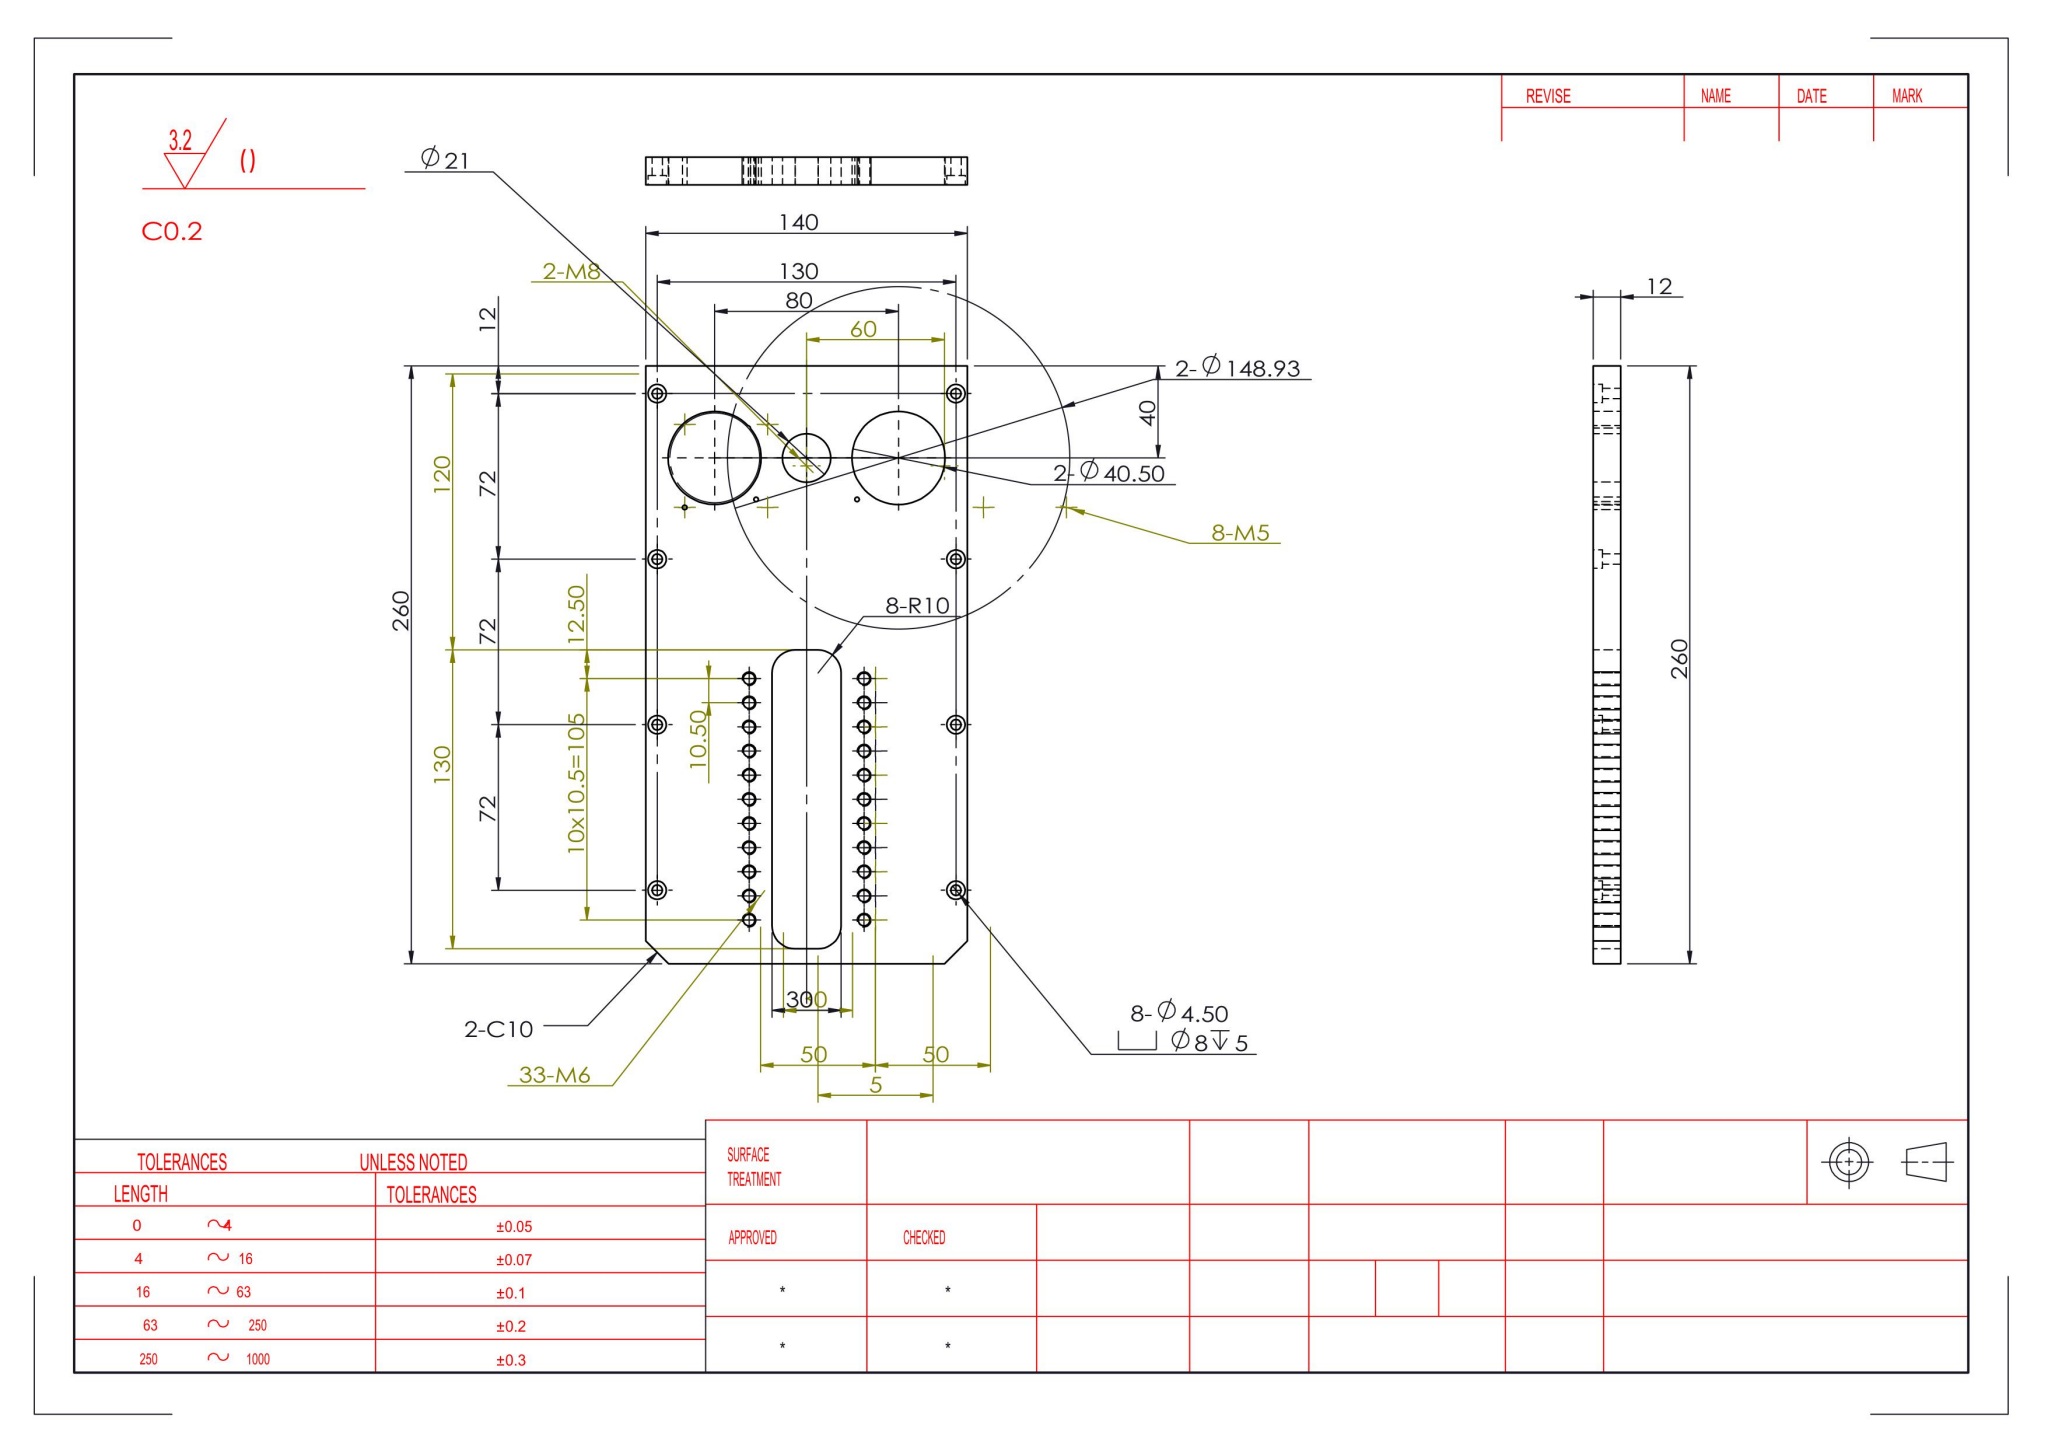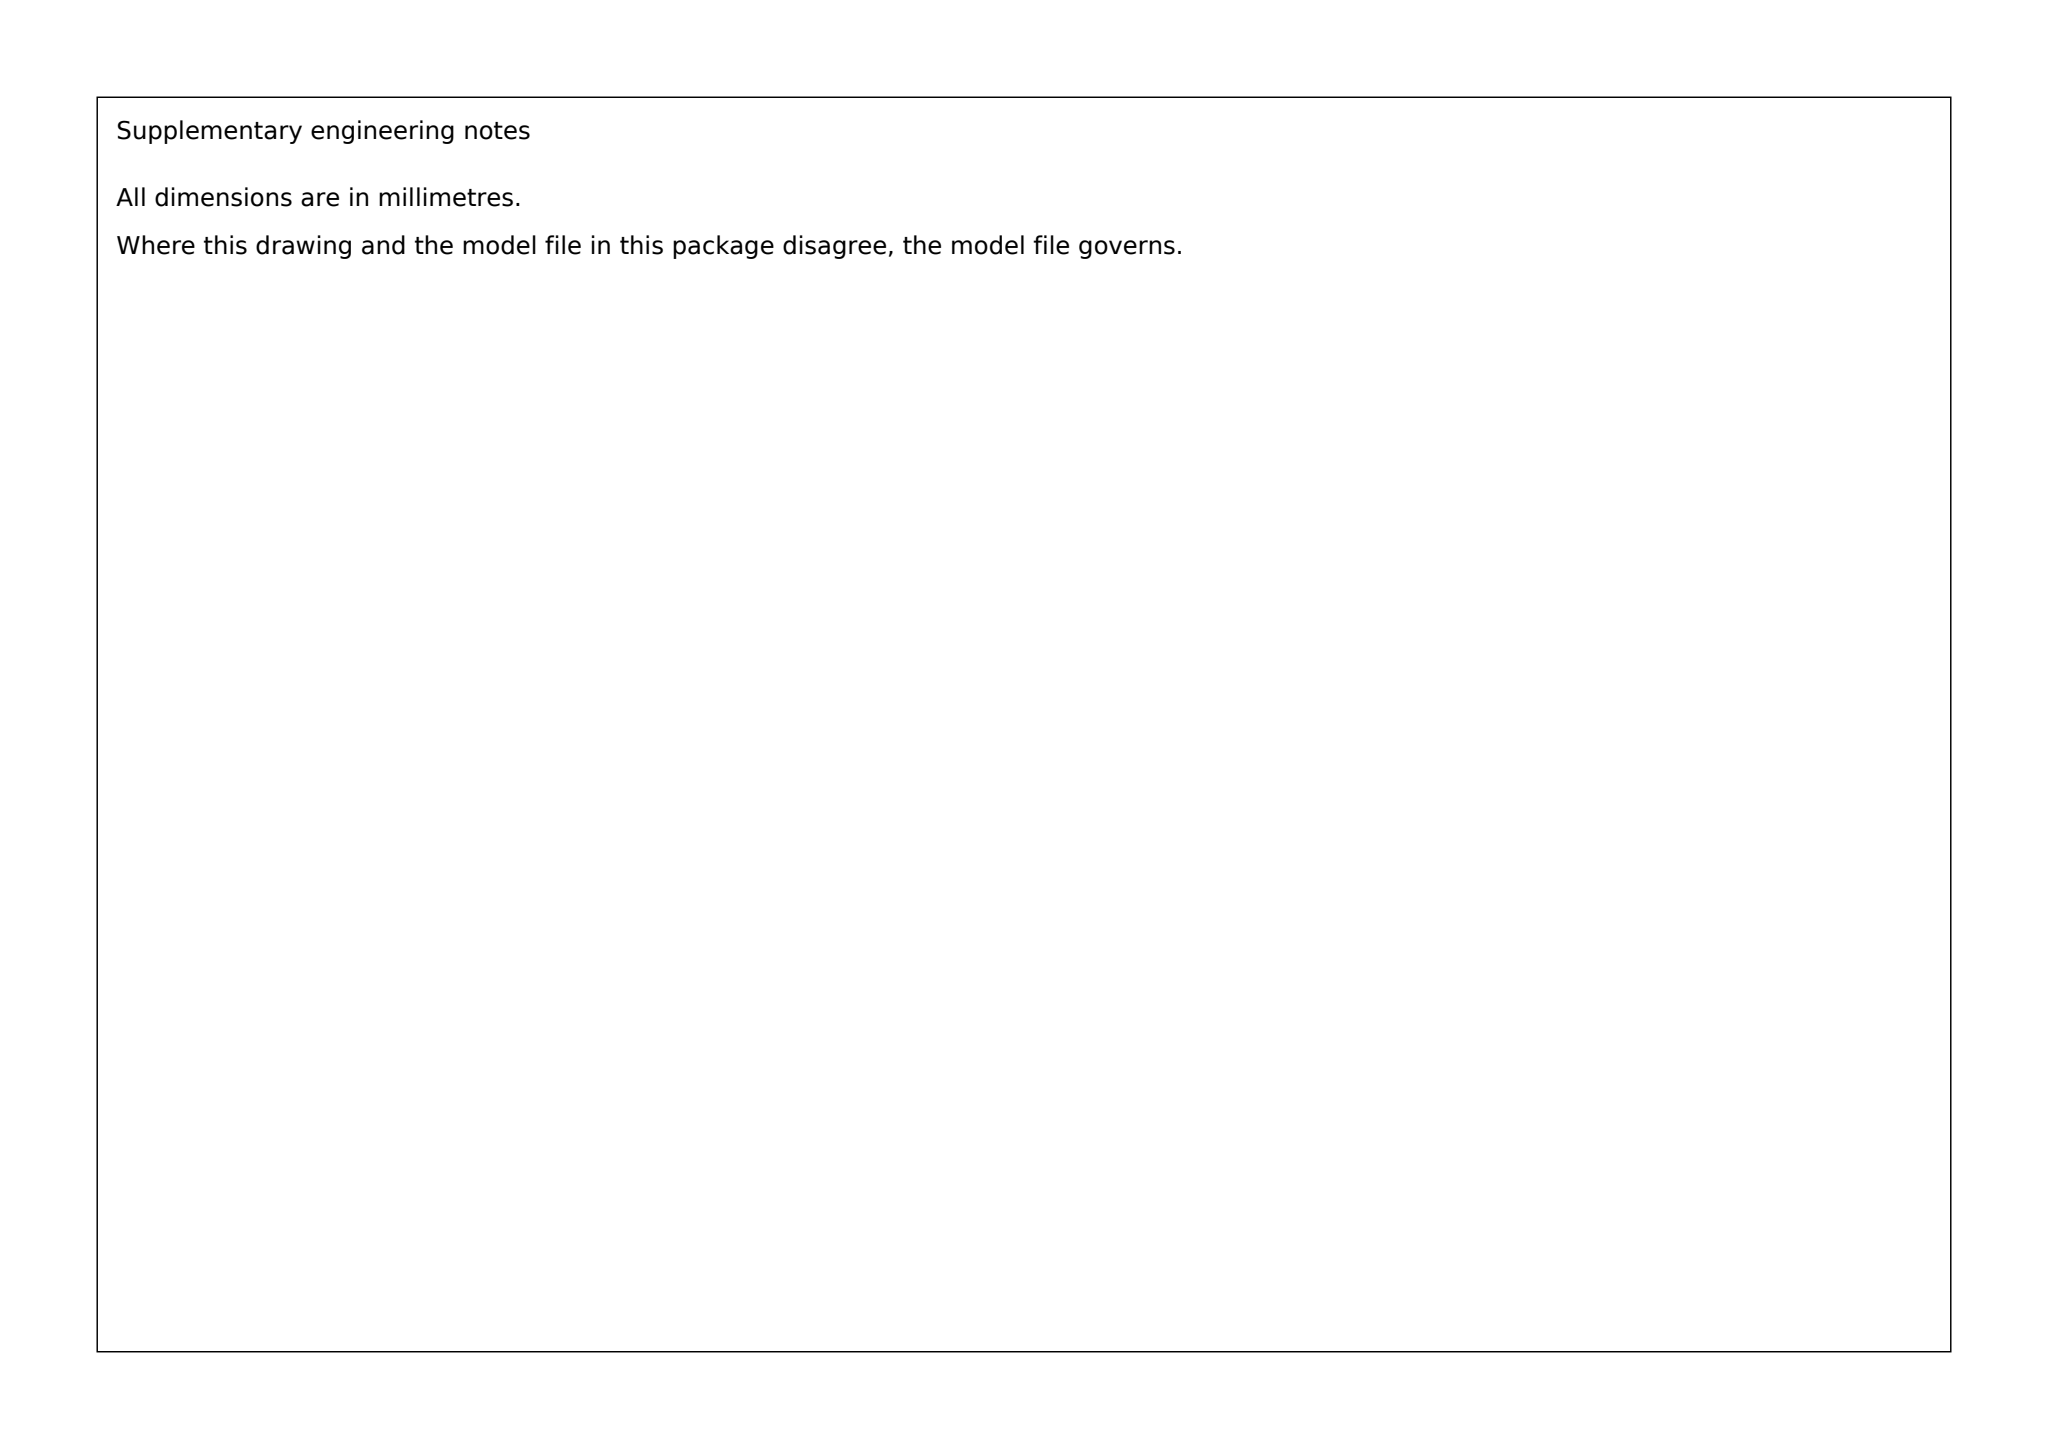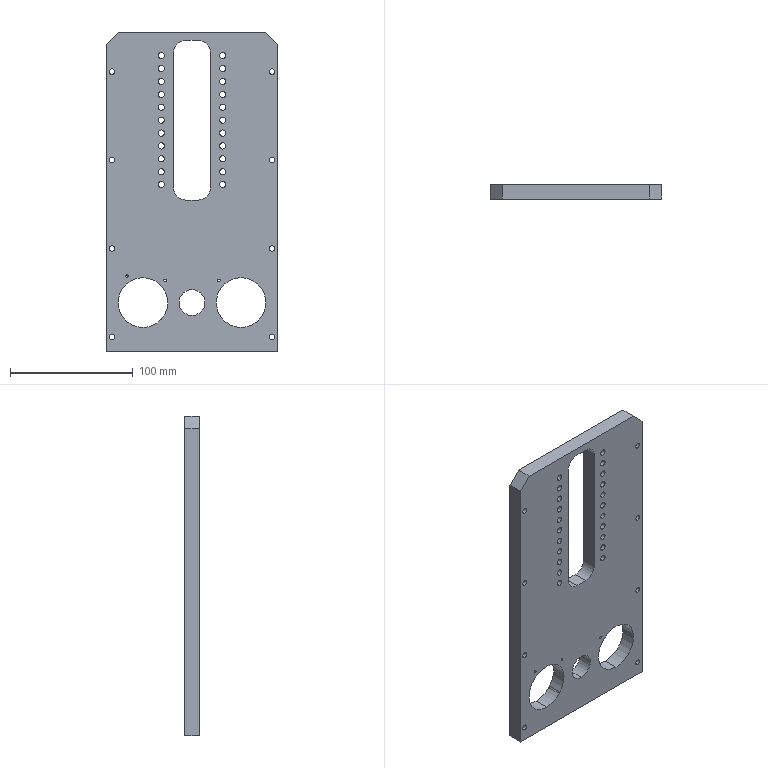Part | SolidWorks | mm | 1 solid | 114 faces | box 140 x 12 x 260 mm | volume 346829 mm3 | cylinder 94 | plane 20 | commonest cylinder face diameters 5 x44 8 x16 4.5 x16 2 x7 40.5 x5 20 x4 21 x2
build123d program:
from build123d import *

# Parameters (mm, degrees)
SKETCH1_W                                       = 140
SKETCH1_H                                       = 260
SKETCH1_R                                       = 20.25
SKETCH1_R_2                                     = 10.5
SKETCH1_W_2                                     = 30
SKETCH1_H_2                                     = 130
EXTRUDE1_DEPTH                                  = 12
CHAMFER1_SIZE                                   = 10
FILLET1_R                                       = 10
M6_TAPPED_HOLE1_D                               = 5
M4_HEX_SOCKET_HEAD_CAP_SCREW_CBORE1_D           = 4.5
M4_HEX_SOCKET_HEAD_CAP_SCREW_CBORE1_CBORE_D     = 8
M4_HEX_SOCKET_HEAD_CAP_SCREW_CBORE1_CBORE_DEPTH = 4
SKETCH5_R                                       = 1
EXTRUDE3_DEPTH                                  = 325.49


with BuildPart() as part:
    # Sketch1 → Extrude1 (new body)
    with BuildSketch(Plane(origin=(0, 0, 0), x_dir=(1, 0, 0), z_dir=(0, 1, 0))):
        with Locations((-19.315, 181.726)):
            Rectangle(SKETCH1_W, SKETCH1_H)
        with Locations(Location((-59.315, 271.726, 0), (0, 0, 270))):
            Circle(SKETCH1_R, mode=Mode.SUBTRACT)
        with Locations(Location((20.685, 271.726, 0), (0, 0, 270))):
            Circle(SKETCH1_R, mode=Mode.SUBTRACT)
        with Locations(Location((-19.315, 271.726, 0), (0, 0, 270))):
            Circle(SKETCH1_R_2, mode=Mode.SUBTRACT)
        with Locations((-19.315, 123.242)):
            Rectangle(SKETCH1_W_2, SKETCH1_H_2, mode=Mode.SUBTRACT)
    extrude(amount=EXTRUDE1_DEPTH)

    # Chamfer1
    chamfer1_edges = [part.edges().sort_by_distance(p)[0] for p in [
        (50.685, 6, -51.726),
        (-89.315, 6, -51.726),
    ]]
    chamfer(chamfer1_edges, length=CHAMFER1_SIZE)

    # Fillet1
    fillet1_edges = [part.edges().sort_by_distance(p)[0] for p in [
        (-34.315, 6, -58.242),
        (-4.315, 6, -58.242),
        (-4.315, 6, -188.242),
        (-34.315, 6, -188.242),
    ]]
    fillet(fillet1_edges, radius=FILLET1_R)

    # M6 Tapped Hole1 (through all)
    with Locations(Plane(origin=(5.685, 12, -70.742), x_dir=(0, 0, 1), z_dir=(0, 1, 0))):
        with Locations((0, 0), (-21, -50), (-42, 0), (-84, 0), (-105, -50), (-63, -50), (-84, -50), (-42, -50), (0, -50), (-21, 0), (-63, 0), (-105, 0), (-94.5, -50), (-73.5, -50), (-52.5, -50), (-31.5, -50), (-10.5, -50), (-94.5, 0), (-73.5, 0), (-52.5, 0), (-31.5, 0), (-10.5, 0)):
            Hole(M6_TAPPED_HOLE1_D / 2)

    # M4 Hex Socket Head Cap Screw CBORE1 (through all)
    with Locations(Plane(origin=(-84.315, 12, -299.726), x_dir=(0, 0, 1), z_dir=(0, 1, 0))):
        with Locations((0, 0), (72, 0), (144, 0), (216, 0), (0, 130), (72, 130), (144, 130), (216, 130)):
            CounterBoreHole(M4_HEX_SOCKET_HEAD_CAP_SCREW_CBORE1_D / 2, M4_HEX_SOCKET_HEAD_CAP_SCREW_CBORE1_CBORE_D / 2, M4_HEX_SOCKET_HEAD_CAP_SCREW_CBORE1_CBORE_DEPTH)

    # Sketch5 → Extrude3 (cut, through all)
    with BuildSketch(Plane(origin=(0, 12, 0), x_dir=(-1, 0, 0), z_dir=(0, 1, 0))):
        with Locations(Location((41.284, -253.694, 0), (0, 0, 90))):
            Circle(SKETCH5_R)
        with Locations(Location((-2.654, -253.694, 0), (0, 0, 90))):
            Circle(SKETCH5_R)
        with Locations(Location((72.346, -250.211, 0), (0, 0, 90))):
            Circle(SKETCH5_R)
        with Locations((75.83, -281.273)):
            Circle(SKETCH5_R)
        with Locations((44.767, -284.757)):
            Circle(SKETCH5_R)
    extrude(amount=-EXTRUDE3_DEPTH, mode=Mode.SUBTRACT)


solid = part.part